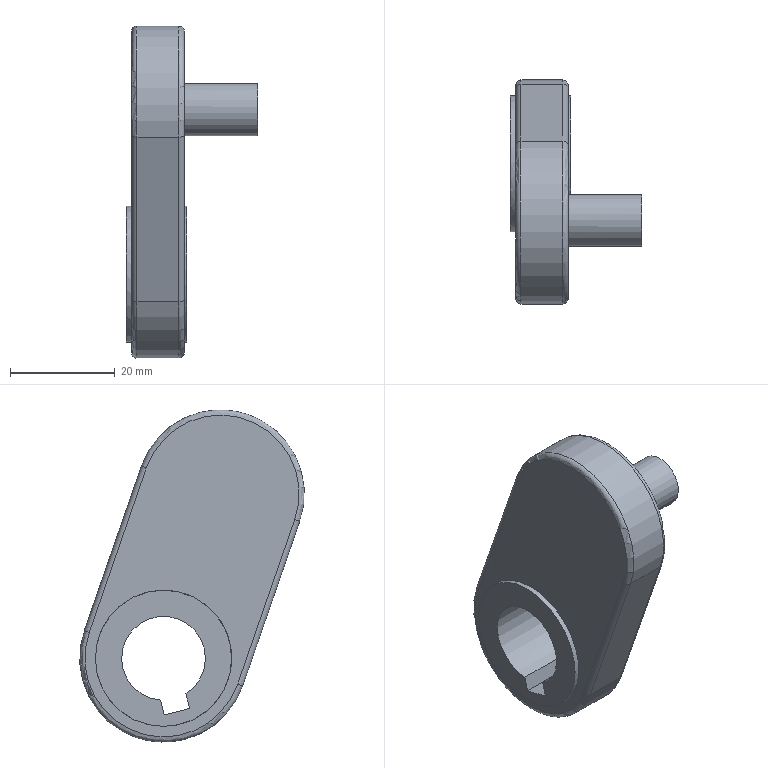Component | NX | CRANK | 1 solid | 24 faces | volume 18041 mm3 | plane 10 | cylinder 10 | torus 4 | commonest cylinder face diameters 2 x4 32 x2 26 x2 10 x1 16 x1